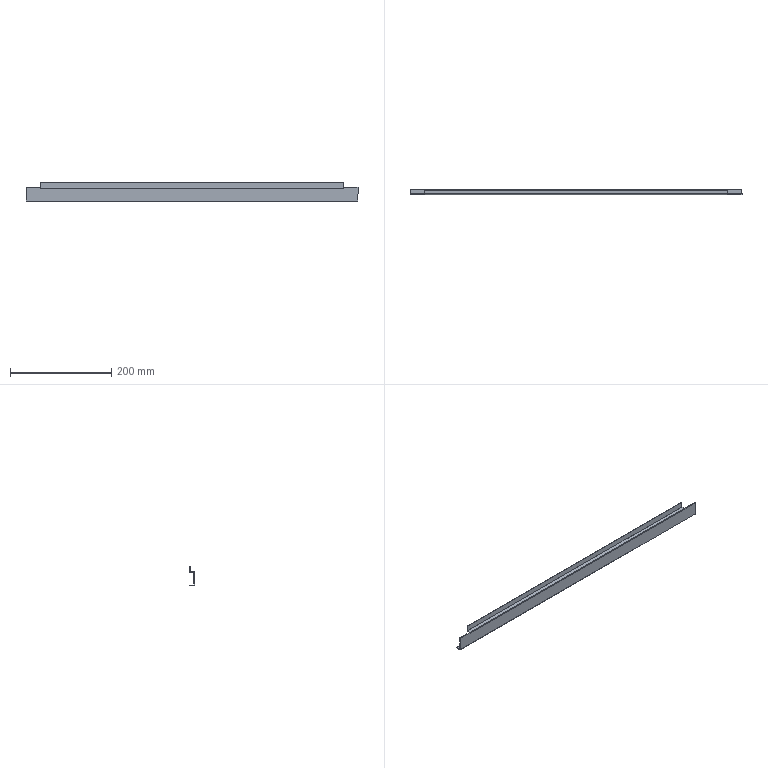Component | SolidWorks | TopCoverRearSideBeam-1 | 1 solid | 40 faces | box 657 x 10 x 39 mm | volume 52545 mm3 | plane 34 | cylinder 6 | commonest cylinder face diameters 0.2 x3 3.2 x3
STEP:
#1=CARTESIAN_POINT('',(10.065,14.168,24.67));
#2=VERTEX_POINT('',#1);
#3=CARTESIAN_POINT('',(10.065,14.168,24.675));
#4=VERTEX_POINT('',#3);
#5=CARTESIAN_POINT('',(10.065,14.168,24.675));
#6=DIRECTION('',(0.,0.,1.));
#7=VECTOR('',#6,39.37);
#8=LINE('',#5,#7);
#9=EDGE_CURVE('',#2,#4,#8,.T.);
#10=ORIENTED_EDGE('',*,*,#9,.F.);
#11=CARTESIAN_POINT('',(10.065,14.164,24.671));
#12=VERTEX_POINT('',#11);
#13=CARTESIAN_POINT('',(10.065,14.164,24.67));
#14=DIRECTION('',(-0.,-1.,0.));
#15=VECTOR('',#14,39.37);
#16=LINE('',#13,#15);
#17=EDGE_CURVE('',#2,#12,#16,.T.);
#18=ORIENTED_EDGE('',*,*,#17,.T.);
#19=CARTESIAN_POINT('',(10.065,14.164,24.612));
#20=VERTEX_POINT('',#19);
#21=CARTESIAN_POINT('',(10.065,14.164,24.671));
#22=DIRECTION('',(-0.,-0.,-1.));
#23=VECTOR('',#22,39.37);
#24=LINE('',#21,#23);
#25=EDGE_CURVE('',#12,#20,#24,.T.);
#26=ORIENTED_EDGE('',*,*,#25,.T.);
#27=CARTESIAN_POINT('',(10.065,14.227,24.675));
#28=VERTEX_POINT('',#27);
#29=CARTESIAN_POINT('',(10.065,14.164,24.675));
#30=DIRECTION('',(1.,-0.,-0.));
#31=DIRECTION('',(0.,1.,0.));
#32=AXIS2_PLACEMENT_3D('',#29,#30,#31);
#33=CIRCLE('',#32,0.06299);
#34=EDGE_CURVE('',#20,#28,#33,.T.);
#35=ORIENTED_EDGE('',*,*,#34,.T.);
#36=CARTESIAN_POINT('',(10.065,14.227,24.675));
#37=DIRECTION('',(0.,1.,-0.));
#38=VECTOR('',#37,39.37);
#39=LINE('',#36,#38);
#40=EDGE_CURVE('',#4,#28,#39,.T.);
#41=ORIENTED_EDGE('',*,*,#40,.F.);
#42=EDGE_LOOP('',(#10,#18,#26,#35,#41));
#43=FACE_OUTER_BOUND('',#42,.T.);
#44=CARTESIAN_POINT('',(10.065,14.164,24.675));
#45=DIRECTION('',(1.,-0.,-0.));
#46=DIRECTION('',(-0.,-1.,0.));
#47=AXIS2_PLACEMENT_3D('',#44,#45,#46);
#48=PLANE('',#47);
#49=ADVANCED_FACE('',(#43),#48,.T.);
#50=CARTESIAN_POINT('',(-13.557,14.164,24.671));
#51=VERTEX_POINT('',#50);
#52=CARTESIAN_POINT('',(-13.557,14.164,24.612));
#53=VERTEX_POINT('',#52);
#54=CARTESIAN_POINT('',(-13.557,14.164,24.671));
#55=DIRECTION('',(-0.,-0.,-1.));
#56=VECTOR('',#55,39.37);
#57=LINE('',#54,#56);
#58=EDGE_CURVE('',#51,#53,#57,.T.);
#59=ORIENTED_EDGE('',*,*,#58,.F.);
#60=CARTESIAN_POINT('',(-13.557,14.168,24.67));
#61=VERTEX_POINT('',#60);
#62=CARTESIAN_POINT('',(-13.557,14.164,24.67));
#63=DIRECTION('',(0.,1.,-0.));
#64=VECTOR('',#63,39.37);
#65=LINE('',#62,#64);
#66=EDGE_CURVE('',#51,#61,#65,.T.);
#67=ORIENTED_EDGE('',*,*,#66,.T.);
#68=CARTESIAN_POINT('',(-13.557,14.168,24.675));
#69=VERTEX_POINT('',#68);
#70=CARTESIAN_POINT('',(-13.557,14.168,24.675));
#71=DIRECTION('',(-0.,-0.,-1.));
#72=VECTOR('',#71,39.37);
#73=LINE('',#70,#72);
#74=EDGE_CURVE('',#69,#61,#73,.T.);
#75=ORIENTED_EDGE('',*,*,#74,.F.);
#76=CARTESIAN_POINT('',(-13.557,14.227,24.675));
#77=VERTEX_POINT('',#76);
#78=CARTESIAN_POINT('',(-13.557,14.168,24.675));
#79=DIRECTION('',(0.,1.,-0.));
#80=VECTOR('',#79,39.37);
#81=LINE('',#78,#80);
#82=EDGE_CURVE('',#69,#77,#81,.T.);
#83=ORIENTED_EDGE('',*,*,#82,.T.);
#84=CARTESIAN_POINT('',(-13.557,14.164,24.675));
#85=DIRECTION('',(-1.,0.,0.));
#86=DIRECTION('',(0.,1.,0.));
#87=AXIS2_PLACEMENT_3D('',#84,#85,#86);
#88=CIRCLE('',#87,0.06299);
#89=EDGE_CURVE('',#77,#53,#88,.T.);
#90=ORIENTED_EDGE('',*,*,#89,.T.);
#91=EDGE_LOOP('',(#59,#67,#75,#83,#90));
#92=FACE_OUTER_BOUND('',#91,.T.);
#93=CARTESIAN_POINT('',(-13.557,14.164,24.675));
#94=DIRECTION('',(1.,-0.,-0.));
#95=DIRECTION('',(-0.,-1.,0.));
#96=AXIS2_PLACEMENT_3D('',#93,#94,#95);
#97=PLANE('',#96);
#98=ADVANCED_FACE('',(#92),#97,.F.);
#99=CARTESIAN_POINT('',(9.982,14.168,24.675));
#100=VERTEX_POINT('',#99);
#101=CARTESIAN_POINT('',(9.982,14.164,24.671));
#102=VERTEX_POINT('',#101);
#103=CARTESIAN_POINT('',(9.982,14.164,24.675));
#104=DIRECTION('',(-1.,0.,0.));
#105=DIRECTION('',(0.,-1.,0.));
#106=AXIS2_PLACEMENT_3D('',#103,#104,#105);
#107=CIRCLE('',#106,0.003937);
#108=EDGE_CURVE('',#100,#102,#107,.T.);
#109=ORIENTED_EDGE('',*,*,#108,.F.);
#110=CARTESIAN_POINT('',(-13.475,14.168,24.675));
#111=VERTEX_POINT('',#110);
#112=CARTESIAN_POINT('',(10.065,14.168,24.675));
#113=DIRECTION('',(-1.,0.,0.));
#114=VECTOR('',#113,39.37);
#115=LINE('',#112,#114);
#116=EDGE_CURVE('',#100,#111,#115,.T.);
#117=ORIENTED_EDGE('',*,*,#116,.T.);
#118=CARTESIAN_POINT('',(-13.475,14.164,24.671));
#119=VERTEX_POINT('',#118);
#120=CARTESIAN_POINT('',(-13.475,14.164,24.675));
#121=DIRECTION('',(1.,-0.,-0.));
#122=DIRECTION('',(0.,1.,-0.));
#123=AXIS2_PLACEMENT_3D('',#120,#121,#122);
#124=CIRCLE('',#123,0.003937);
#125=EDGE_CURVE('',#119,#111,#124,.T.);
#126=ORIENTED_EDGE('',*,*,#125,.F.);
#127=CARTESIAN_POINT('',(-13.557,14.164,24.671));
#128=DIRECTION('',(1.,-0.,-0.));
#129=VECTOR('',#128,39.37);
#130=LINE('',#127,#129);
#131=EDGE_CURVE('',#119,#102,#130,.T.);
#132=ORIENTED_EDGE('',*,*,#131,.T.);
#133=EDGE_LOOP('',(#109,#117,#126,#132));
#134=FACE_OUTER_BOUND('',#133,.T.);
#135=CARTESIAN_POINT('',(-13.557,14.164,24.675));
#136=DIRECTION('',(-1.,0.,0.));
#137=DIRECTION('',(0.,1.,0.));
#138=AXIS2_PLACEMENT_3D('',#135,#136,#137);
#139=CYLINDRICAL_SURFACE('',#138,0.003937);
#140=ADVANCED_FACE('',(#134),#139,.F.);
#141=ORIENTED_EDGE('',*,*,#58,.T.);
#142=CARTESIAN_POINT('',(-13.557,13.896,24.612));
#143=VERTEX_POINT('',#142);
#144=CARTESIAN_POINT('',(-13.557,13.892,24.612));
#145=DIRECTION('',(-0.,-1.,-0.));
#146=VECTOR('',#145,39.37);
#147=LINE('',#144,#146);
#148=EDGE_CURVE('',#53,#143,#147,.T.);
#149=ORIENTED_EDGE('',*,*,#148,.T.);
#150=CARTESIAN_POINT('',(-13.557,13.896,24.671));
#151=VERTEX_POINT('',#150);
#152=CARTESIAN_POINT('',(-13.557,13.896,24.671));
#153=DIRECTION('',(0.,-0.,1.));
#154=VECTOR('',#153,39.37);
#155=LINE('',#152,#154);
#156=EDGE_CURVE('',#143,#151,#155,.T.);
#157=ORIENTED_EDGE('',*,*,#156,.T.);
#158=CARTESIAN_POINT('',(-13.557,13.892,24.671));
#159=DIRECTION('',(-0.,-1.,-0.));
#160=VECTOR('',#159,39.37);
#161=LINE('',#158,#160);
#162=EDGE_CURVE('',#51,#151,#161,.T.);
#163=ORIENTED_EDGE('',*,*,#162,.F.);
#164=EDGE_LOOP('',(#141,#149,#157,#163));
#165=FACE_OUTER_BOUND('',#164,.T.);
#166=CARTESIAN_POINT('',(-13.557,13.892,24.671));
#167=DIRECTION('',(1.,-0.,-0.));
#168=DIRECTION('',(-0.,-1.,0.));
#169=AXIS2_PLACEMENT_3D('',#166,#167,#168);
#170=PLANE('',#169);
#171=ADVANCED_FACE('',(#165),#170,.F.);
#172=ORIENTED_EDGE('',*,*,#25,.F.);
#173=CARTESIAN_POINT('',(10.065,13.896,24.671));
#174=VERTEX_POINT('',#173);
#175=CARTESIAN_POINT('',(10.065,13.892,24.671));
#176=DIRECTION('',(0.,1.,0.));
#177=VECTOR('',#176,39.37);
#178=LINE('',#175,#177);
#179=EDGE_CURVE('',#174,#12,#178,.T.);
#180=ORIENTED_EDGE('',*,*,#179,.F.);
#181=CARTESIAN_POINT('',(10.065,13.896,24.612));
#182=VERTEX_POINT('',#181);
#183=CARTESIAN_POINT('',(10.065,13.896,24.612));
#184=DIRECTION('',(0.,-0.,1.));
#185=VECTOR('',#184,39.37);
#186=LINE('',#183,#185);
#187=EDGE_CURVE('',#182,#174,#186,.T.);
#188=ORIENTED_EDGE('',*,*,#187,.F.);
#189=CARTESIAN_POINT('',(10.065,14.227,24.612));
#190=DIRECTION('',(0.,1.,0.));
#191=VECTOR('',#190,39.37);
#192=LINE('',#189,#191);
#193=EDGE_CURVE('',#182,#20,#192,.T.);
#194=ORIENTED_EDGE('',*,*,#193,.T.);
#195=EDGE_LOOP('',(#172,#180,#188,#194));
#196=FACE_OUTER_BOUND('',#195,.T.);
#197=CARTESIAN_POINT('',(10.065,14.227,24.671));
#198=DIRECTION('',(-1.,0.,0.));
#199=DIRECTION('',(0.,1.,-0.));
#200=AXIS2_PLACEMENT_3D('',#197,#198,#199);
#201=PLANE('',#200);
#202=ADVANCED_FACE('',(#196),#201,.F.);
#203=ORIENTED_EDGE('',*,*,#162,.T.);
#204=CARTESIAN_POINT('',(-13.557,13.896,24.671));
#205=DIRECTION('',(-1.,0.,0.));
#206=VECTOR('',#205,39.37);
#207=LINE('',#204,#206);
#208=EDGE_CURVE('',#174,#151,#207,.T.);
#209=ORIENTED_EDGE('',*,*,#208,.F.);
#210=ORIENTED_EDGE('',*,*,#179,.T.);
#211=CARTESIAN_POINT('',(9.982,14.164,24.671));
#212=CARTESIAN_POINT('',(10.009,14.164,24.67));
#213=CARTESIAN_POINT('',(10.037,14.164,24.67));
#214=CARTESIAN_POINT('',(10.065,14.164,24.671));
#215=B_SPLINE_CURVE_WITH_KNOTS('',3,(#211,#212,#213,#214),.UNSPECIFIED.,.F.,.F.,(4,4),(0.9965,1.),.UNSPECIFIED.);
#216=EDGE_CURVE('',#102,#12,#215,.T.);
#217=ORIENTED_EDGE('',*,*,#216,.F.);
#218=ORIENTED_EDGE('',*,*,#131,.F.);
#219=CARTESIAN_POINT('',(-13.557,14.164,24.671));
#220=CARTESIAN_POINT('',(-13.53,14.164,24.67));
#221=CARTESIAN_POINT('',(-13.502,14.164,24.67));
#222=CARTESIAN_POINT('',(-13.475,14.164,24.671));
#223=B_SPLINE_CURVE_WITH_KNOTS('',3,(#219,#220,#221,#222),.UNSPECIFIED.,.F.,.F.,(4,4),(0.,0.0035),.UNSPECIFIED.);
#224=EDGE_CURVE('',#51,#119,#223,.T.);
#225=ORIENTED_EDGE('',*,*,#224,.F.);
#226=EDGE_LOOP('',(#203,#209,#210,#217,#218,#225));
#227=FACE_OUTER_BOUND('',#226,.T.);
#228=CARTESIAN_POINT('',(-1.746,13.892,24.671));
#229=DIRECTION('',(-0.,0.,-1.));
#230=DIRECTION('',(0.,1.,0.));
#231=AXIS2_PLACEMENT_3D('',#228,#229,#230);
#232=PLANE('',#231);
#233=ADVANCED_FACE('',(#227),#232,.F.);
#234=ORIENTED_EDGE('',*,*,#148,.F.);
#235=CARTESIAN_POINT('',(-13.557,14.164,24.612));
#236=DIRECTION('',(1.,-0.,-0.));
#237=VECTOR('',#236,39.37);
#238=LINE('',#235,#237);
#239=EDGE_CURVE('',#53,#20,#238,.T.);
#240=ORIENTED_EDGE('',*,*,#239,.T.);
#241=ORIENTED_EDGE('',*,*,#193,.F.);
#242=CARTESIAN_POINT('',(-13.557,13.896,24.612));
#243=DIRECTION('',(1.,-0.,-0.));
#244=VECTOR('',#243,39.37);
#245=LINE('',#242,#244);
#246=EDGE_CURVE('',#143,#182,#245,.T.);
#247=ORIENTED_EDGE('',*,*,#246,.F.);
#248=EDGE_LOOP('',(#234,#240,#241,#247));
#249=FACE_OUTER_BOUND('',#248,.T.);
#250=CARTESIAN_POINT('',(-1.746,13.892,24.612));
#251=DIRECTION('',(-0.,0.,-1.));
#252=DIRECTION('',(0.,1.,0.));
#253=AXIS2_PLACEMENT_3D('',#250,#251,#252);
#254=PLANE('',#253);
#255=ADVANCED_FACE('',(#249),#254,.T.);
#256=CARTESIAN_POINT('',(-14.68,13.833,23.612));
#257=VERTEX_POINT('',#256);
#258=CARTESIAN_POINT('',(-14.68,13.833,24.671));
#259=VERTEX_POINT('',#258);
#260=CARTESIAN_POINT('',(-14.68,13.833,24.671));
#261=DIRECTION('',(0.,0.,1.));
#262=VECTOR('',#261,39.37);
#263=LINE('',#260,#262);
#264=EDGE_CURVE('',#257,#259,#263,.T.);
#265=ORIENTED_EDGE('',*,*,#264,.F.);
#266=CARTESIAN_POINT('',(11.187,13.833,23.612));
#267=VERTEX_POINT('',#266);
#268=CARTESIAN_POINT('',(-14.68,13.833,23.612));
#269=DIRECTION('',(1.,-0.,-0.));
#270=VECTOR('',#269,39.37);
#271=LINE('',#268,#270);
#272=EDGE_CURVE('',#257,#267,#271,.T.);
#273=ORIENTED_EDGE('',*,*,#272,.T.);
#274=CARTESIAN_POINT('',(11.187,13.833,24.671));
#275=VERTEX_POINT('',#274);
#276=CARTESIAN_POINT('',(11.187,13.833,24.671));
#277=DIRECTION('',(-0.,-0.,-1.));
#278=VECTOR('',#277,39.37);
#279=LINE('',#276,#278);
#280=EDGE_CURVE('',#275,#267,#279,.T.);
#281=ORIENTED_EDGE('',*,*,#280,.F.);
#282=CARTESIAN_POINT('',(10.065,13.833,24.671));
#283=VERTEX_POINT('',#282);
#284=CARTESIAN_POINT('',(-14.68,13.833,24.671));
#285=DIRECTION('',(1.,-0.,-0.));
#286=VECTOR('',#285,39.37);
#287=LINE('',#284,#286);
#288=EDGE_CURVE('',#283,#275,#287,.T.);
#289=ORIENTED_EDGE('',*,*,#288,.F.);
#290=CARTESIAN_POINT('',(10.065,13.833,24.608));
#291=VERTEX_POINT('',#290);
#292=CARTESIAN_POINT('',(10.065,13.833,24.11));
#293=DIRECTION('',(-0.,-0.,-1.));
#294=VECTOR('',#293,39.37);
#295=LINE('',#292,#294);
#296=EDGE_CURVE('',#283,#291,#295,.T.);
#297=ORIENTED_EDGE('',*,*,#296,.T.);
#298=CARTESIAN_POINT('',(-13.557,13.833,24.608));
#299=VERTEX_POINT('',#298);
#300=CARTESIAN_POINT('',(10.065,13.833,24.608));
#301=DIRECTION('',(-1.,0.,0.));
#302=VECTOR('',#301,39.37);
#303=LINE('',#300,#302);
#304=EDGE_CURVE('',#291,#299,#303,.T.);
#305=ORIENTED_EDGE('',*,*,#304,.T.);
#306=CARTESIAN_POINT('',(-13.557,13.833,24.671));
#307=VERTEX_POINT('',#306);
#308=CARTESIAN_POINT('',(-13.557,13.833,24.11));
#309=DIRECTION('',(0.,0.,1.));
#310=VECTOR('',#309,39.37);
#311=LINE('',#308,#310);
#312=EDGE_CURVE('',#299,#307,#311,.T.);
#313=ORIENTED_EDGE('',*,*,#312,.T.);
#314=CARTESIAN_POINT('',(-14.68,13.833,24.671));
#315=DIRECTION('',(1.,-0.,-0.));
#316=VECTOR('',#315,39.37);
#317=LINE('',#314,#316);
#318=EDGE_CURVE('',#259,#307,#317,.T.);
#319=ORIENTED_EDGE('',*,*,#318,.F.);
#320=EDGE_LOOP('',(#265,#273,#281,#289,#297,#305,#313,#319));
#321=FACE_OUTER_BOUND('',#320,.T.);
#322=CARTESIAN_POINT('',(-1.746,13.833,24.11));
#323=DIRECTION('',(-0.,-1.,0.));
#324=DIRECTION('',(-1.,0.,0.));
#325=AXIS2_PLACEMENT_3D('',#322,#323,#324);
#326=PLANE('',#325);
#327=ADVANCED_FACE('',(#321),#326,.T.);
#328=CARTESIAN_POINT('',(-14.68,13.892,23.612));
#329=VERTEX_POINT('',#328);
#330=CARTESIAN_POINT('',(11.187,13.892,23.612));
#331=VERTEX_POINT('',#330);
#332=CARTESIAN_POINT('',(-14.68,13.892,23.612));
#333=DIRECTION('',(1.,-0.,-0.));
#334=VECTOR('',#333,39.37);
#335=LINE('',#332,#334);
#336=EDGE_CURVE('',#329,#331,#335,.T.);
#337=ORIENTED_EDGE('',*,*,#336,.F.);
#338=CARTESIAN_POINT('',(-14.68,13.892,24.671));
#339=VERTEX_POINT('',#338);
#340=CARTESIAN_POINT('',(-14.68,13.892,24.671));
#341=DIRECTION('',(0.,0.,1.));
#342=VECTOR('',#341,39.37);
#343=LINE('',#340,#342);
#344=EDGE_CURVE('',#329,#339,#343,.T.);
#345=ORIENTED_EDGE('',*,*,#344,.T.);
#346=CARTESIAN_POINT('',(-13.557,13.892,24.671));
#347=VERTEX_POINT('',#346);
#348=CARTESIAN_POINT('',(-14.68,13.892,24.671));
#349=DIRECTION('',(1.,-0.,-0.));
#350=VECTOR('',#349,39.37);
#351=LINE('',#348,#350);
#352=EDGE_CURVE('',#339,#347,#351,.T.);
#353=ORIENTED_EDGE('',*,*,#352,.T.);
#354=CARTESIAN_POINT('',(-13.557,13.892,24.671));
#355=VERTEX_POINT('',#354);
#356=CARTESIAN_POINT('',(-13.557,13.892,24.608));
#357=DIRECTION('',(0.,-0.,1.));
#358=VECTOR('',#357,39.37);
#359=LINE('',#356,#358);
#360=EDGE_CURVE('',#355,#347,#359,.T.);
#361=ORIENTED_EDGE('',*,*,#360,.F.);
#362=CARTESIAN_POINT('',(-13.557,13.892,24.608));
#363=VERTEX_POINT('',#362);
#364=CARTESIAN_POINT('',(-13.557,13.892,24.608));
#365=DIRECTION('',(0.,-0.,1.));
#366=VECTOR('',#365,39.37);
#367=LINE('',#364,#366);
#368=EDGE_CURVE('',#363,#355,#367,.T.);
#369=ORIENTED_EDGE('',*,*,#368,.F.);
#370=CARTESIAN_POINT('',(10.065,13.892,24.608));
#371=VERTEX_POINT('',#370);
#372=CARTESIAN_POINT('',(10.065,13.892,24.608));
#373=DIRECTION('',(-1.,0.,0.));
#374=VECTOR('',#373,39.37);
#375=LINE('',#372,#374);
#376=EDGE_CURVE('',#371,#363,#375,.T.);
#377=ORIENTED_EDGE('',*,*,#376,.F.);
#378=CARTESIAN_POINT('',(10.065,13.892,24.671));
#379=VERTEX_POINT('',#378);
#380=CARTESIAN_POINT('',(10.065,13.892,24.671));
#381=DIRECTION('',(-0.,0.,-1.));
#382=VECTOR('',#381,39.37);
#383=LINE('',#380,#382);
#384=EDGE_CURVE('',#379,#371,#383,.T.);
#385=ORIENTED_EDGE('',*,*,#384,.F.);
#386=CARTESIAN_POINT('',(10.065,13.892,24.671));
#387=VERTEX_POINT('',#386);
#388=CARTESIAN_POINT('',(10.065,13.892,24.671));
#389=DIRECTION('',(-0.,0.,-1.));
#390=VECTOR('',#389,39.37);
#391=LINE('',#388,#390);
#392=EDGE_CURVE('',#387,#379,#391,.T.);
#393=ORIENTED_EDGE('',*,*,#392,.F.);
#394=CARTESIAN_POINT('',(11.187,13.892,24.671));
#395=VERTEX_POINT('',#394);
#396=CARTESIAN_POINT('',(-14.68,13.892,24.671));
#397=DIRECTION('',(1.,-0.,-0.));
#398=VECTOR('',#397,39.37);
#399=LINE('',#396,#398);
#400=EDGE_CURVE('',#387,#395,#399,.T.);
#401=ORIENTED_EDGE('',*,*,#400,.T.);
#402=CARTESIAN_POINT('',(11.187,13.892,24.671));
#403=DIRECTION('',(-0.,-0.,-1.));
#404=VECTOR('',#403,39.37);
#405=LINE('',#402,#404);
#406=EDGE_CURVE('',#395,#331,#405,.T.);
#407=ORIENTED_EDGE('',*,*,#406,.T.);
#408=EDGE_LOOP('',(#337,#345,#353,#361,#369,#377,#385,#393,#401,#407));
#409=FACE_OUTER_BOUND('',#408,.T.);
#410=CARTESIAN_POINT('',(-1.746,13.892,24.11));
#411=DIRECTION('',(-0.,-1.,0.));
#412=DIRECTION('',(-1.,0.,0.));
#413=AXIS2_PLACEMENT_3D('',#410,#411,#412);
#414=PLANE('',#413);
#415=ADVANCED_FACE('',(#409),#414,.F.);
#416=ORIENTED_EDGE('',*,*,#344,.F.);
#417=CARTESIAN_POINT('',(-14.68,13.892,23.612));
#418=DIRECTION('',(-0.,-1.,0.));
#419=VECTOR('',#418,39.37);
#420=LINE('',#417,#419);
#421=EDGE_CURVE('',#329,#257,#420,.T.);
#422=ORIENTED_EDGE('',*,*,#421,.T.);
#423=ORIENTED_EDGE('',*,*,#264,.T.);
#424=CARTESIAN_POINT('',(-14.68,13.833,24.671));
#425=DIRECTION('',(0.,1.,-0.));
#426=VECTOR('',#425,39.37);
#427=LINE('',#424,#426);
#428=EDGE_CURVE('',#259,#339,#427,.T.);
#429=ORIENTED_EDGE('',*,*,#428,.T.);
#430=EDGE_LOOP('',(#416,#422,#423,#429));
#431=FACE_OUTER_BOUND('',#430,.T.);
#432=CARTESIAN_POINT('',(-14.68,13.833,24.671));
#433=DIRECTION('',(-1.,0.,0.));
#434=DIRECTION('',(0.,1.,-0.));
#435=AXIS2_PLACEMENT_3D('',#432,#433,#434);
#436=PLANE('',#435);
#437=ADVANCED_FACE('',(#431),#436,.T.);
#438=ORIENTED_EDGE('',*,*,#392,.T.);
#439=CARTESIAN_POINT('',(10.065,13.896,24.608));
#440=DIRECTION('',(1.,-0.,-0.));
#441=DIRECTION('',(0.,-1.,0.));
#442=AXIS2_PLACEMENT_3D('',#439,#440,#441);
#443=CIRCLE('',#442,0.06299);
#444=EDGE_CURVE('',#379,#291,#443,.T.);
#445=ORIENTED_EDGE('',*,*,#444,.T.);
#446=ORIENTED_EDGE('',*,*,#296,.F.);
#447=CARTESIAN_POINT('',(10.065,13.892,24.671));
#448=DIRECTION('',(-0.,-1.,-0.));
#449=VECTOR('',#448,39.37);
#450=LINE('',#447,#449);
#451=EDGE_CURVE('',#387,#283,#450,.T.);
#452=ORIENTED_EDGE('',*,*,#451,.F.);
#453=EDGE_LOOP('',(#438,#445,#446,#452));
#454=FACE_OUTER_BOUND('',#453,.T.);
#455=CARTESIAN_POINT('',(10.065,13.892,24.671));
#456=DIRECTION('',(-1.,0.,0.));
#457=DIRECTION('',(0.,1.,-0.));
#458=AXIS2_PLACEMENT_3D('',#455,#456,#457);
#459=PLANE('',#458);
#460=ADVANCED_FACE('',(#454),#459,.T.);
#461=ORIENTED_EDGE('',*,*,#312,.F.);
#462=CARTESIAN_POINT('',(-13.557,13.896,24.608));
#463=DIRECTION('',(-1.,0.,0.));
#464=DIRECTION('',(0.,-1.,0.));
#465=AXIS2_PLACEMENT_3D('',#462,#463,#464);
#466=CIRCLE('',#465,0.06299);
#467=EDGE_CURVE('',#299,#355,#466,.T.);
#468=ORIENTED_EDGE('',*,*,#467,.T.);
#469=ORIENTED_EDGE('',*,*,#360,.T.);
#470=CARTESIAN_POINT('',(-13.557,13.892,24.671));
#471=DIRECTION('',(-0.,-1.,-0.));
#472=VECTOR('',#471,39.37);
#473=LINE('',#470,#472);
#474=EDGE_CURVE('',#347,#307,#473,.T.);
#475=ORIENTED_EDGE('',*,*,#474,.T.);
#476=EDGE_LOOP('',(#461,#468,#469,#475));
#477=FACE_OUTER_BOUND('',#476,.T.);
#478=CARTESIAN_POINT('',(-13.557,13.892,24.608));
#479=DIRECTION('',(1.,-0.,-0.));
#480=DIRECTION('',(-0.,-1.,0.));
#481=AXIS2_PLACEMENT_3D('',#478,#479,#480);
#482=PLANE('',#481);
#483=ADVANCED_FACE('',(#477),#482,.T.);
#484=ORIENTED_EDGE('',*,*,#400,.F.);
#485=ORIENTED_EDGE('',*,*,#451,.T.);
#486=ORIENTED_EDGE('',*,*,#288,.T.);
#487=CARTESIAN_POINT('',(11.187,13.833,24.671));
#488=DIRECTION('',(0.,1.,-0.));
#489=VECTOR('',#488,39.37);
#490=LINE('',#487,#489);
#491=EDGE_CURVE('',#275,#395,#490,.T.);
#492=ORIENTED_EDGE('',*,*,#491,.T.);
#493=EDGE_LOOP('',(#484,#485,#486,#492));
#494=FACE_OUTER_BOUND('',#493,.T.);
#495=CARTESIAN_POINT('',(-14.68,13.833,24.671));
#496=DIRECTION('',(0.,0.,1.));
#497=DIRECTION('',(-0.,-1.,0.));
#498=AXIS2_PLACEMENT_3D('',#495,#496,#497);
#499=PLANE('',#498);
#500=ADVANCED_FACE('',(#494),#499,.T.);
#501=ORIENTED_EDGE('',*,*,#318,.T.);
#502=ORIENTED_EDGE('',*,*,#474,.F.);
#503=ORIENTED_EDGE('',*,*,#352,.F.);
#504=ORIENTED_EDGE('',*,*,#428,.F.);
#505=EDGE_LOOP('',(#501,#502,#503,#504));
#506=FACE_OUTER_BOUND('',#505,.T.);
#507=CARTESIAN_POINT('',(-14.68,13.833,24.671));
#508=DIRECTION('',(0.,0.,1.));
#509=DIRECTION('',(-0.,-1.,0.));
#510=AXIS2_PLACEMENT_3D('',#507,#508,#509);
#511=PLANE('',#510);
#512=ADVANCED_FACE('',(#506),#511,.T.);
#513=CARTESIAN_POINT('',(11.187,13.892,23.612));
#514=DIRECTION('',(-0.,-1.,0.));
#515=VECTOR('',#514,39.37);
#516=LINE('',#513,#515);
#517=EDGE_CURVE('',#331,#267,#516,.T.);
#518=ORIENTED_EDGE('',*,*,#517,.F.);
#519=ORIENTED_EDGE('',*,*,#406,.F.);
#520=ORIENTED_EDGE('',*,*,#491,.F.);
#521=ORIENTED_EDGE('',*,*,#280,.T.);
#522=EDGE_LOOP('',(#518,#519,#520,#521));
#523=FACE_OUTER_BOUND('',#522,.T.);
#524=CARTESIAN_POINT('',(11.187,13.833,24.671));
#525=DIRECTION('',(1.,-0.,-0.));
#526=DIRECTION('',(-0.,-1.,0.));
#527=AXIS2_PLACEMENT_3D('',#524,#525,#526);
#528=PLANE('',#527);
#529=ADVANCED_FACE('',(#523),#528,.T.);
#530=CARTESIAN_POINT('',(-13.557,13.896,24.608));
#531=DIRECTION('',(-1.,0.,0.));
#532=DIRECTION('',(0.,-1.,0.));
#533=AXIS2_PLACEMENT_3D('',#530,#531,#532);
#534=CIRCLE('',#533,0.003937);
#535=EDGE_CURVE('',#363,#143,#534,.T.);
#536=ORIENTED_EDGE('',*,*,#535,.F.);
#537=ORIENTED_EDGE('',*,*,#368,.T.);
#538=CARTESIAN_POINT('',(-13.557,13.896,24.608));
#539=DIRECTION('',(-1.,0.,0.));
#540=DIRECTION('',(0.,-1.,0.));
#541=AXIS2_PLACEMENT_3D('',#538,#539,#540);
#542=CIRCLE('',#541,0.06299);
#543=EDGE_CURVE('',#355,#151,#542,.T.);
#544=ORIENTED_EDGE('',*,*,#543,.T.);
#545=ORIENTED_EDGE('',*,*,#156,.F.);
#546=EDGE_LOOP('',(#536,#537,#544,#545));
#547=FACE_OUTER_BOUND('',#546,.T.);
#548=CARTESIAN_POINT('',(-13.557,13.896,24.608));
#549=DIRECTION('',(-1.,0.,0.));
#550=DIRECTION('',(0.,1.,-0.));
#551=AXIS2_PLACEMENT_3D('',#548,#549,#550);
#552=PLANE('',#551);
#553=ADVANCED_FACE('',(#547),#552,.T.);
#554=CARTESIAN_POINT('',(10.065,13.896,24.608));
#555=DIRECTION('',(1.,-0.,-0.));
#556=DIRECTION('',(0.,-1.,0.));
#557=AXIS2_PLACEMENT_3D('',#554,#555,#556);
#558=CIRCLE('',#557,0.06299);
#559=EDGE_CURVE('',#174,#379,#558,.T.);
#560=ORIENTED_EDGE('',*,*,#559,.T.);
#561=ORIENTED_EDGE('',*,*,#384,.T.);
#562=CARTESIAN_POINT('',(10.065,13.896,24.608));
#563=DIRECTION('',(1.,-0.,-0.));
#564=DIRECTION('',(0.,-1.,0.));
#565=AXIS2_PLACEMENT_3D('',#562,#563,#564);
#566=CIRCLE('',#565,0.003937);
#567=EDGE_CURVE('',#182,#371,#566,.T.);
#568=ORIENTED_EDGE('',*,*,#567,.F.);
#569=ORIENTED_EDGE('',*,*,#187,.T.);
#570=EDGE_LOOP('',(#560,#561,#568,#569));
#571=FACE_OUTER_BOUND('',#570,.T.);
#572=CARTESIAN_POINT('',(10.065,13.896,24.608));
#573=DIRECTION('',(-1.,0.,0.));
#574=DIRECTION('',(0.,1.,-0.));
#575=AXIS2_PLACEMENT_3D('',#572,#573,#574);
#576=PLANE('',#575);
#577=ADVANCED_FACE('',(#571),#576,.F.);
#578=ORIENTED_EDGE('',*,*,#304,.F.);
#579=ORIENTED_EDGE('',*,*,#444,.F.);
#580=ORIENTED_EDGE('',*,*,#559,.F.);
#581=ORIENTED_EDGE('',*,*,#208,.T.);
#582=ORIENTED_EDGE('',*,*,#543,.F.);
#583=ORIENTED_EDGE('',*,*,#467,.F.);
#584=EDGE_LOOP('',(#578,#579,#580,#581,#582,#583));
#585=FACE_OUTER_BOUND('',#584,.T.);
#586=CARTESIAN_POINT('',(10.065,13.896,24.608));
#587=DIRECTION('',(1.,-0.,-0.));
#588=DIRECTION('',(0.,0.,1.));
#589=AXIS2_PLACEMENT_3D('',#586,#587,#588);
#590=CYLINDRICAL_SURFACE('',#589,0.06299);
#591=ADVANCED_FACE('',(#585),#590,.T.);
#592=ORIENTED_EDGE('',*,*,#376,.T.);
#593=ORIENTED_EDGE('',*,*,#535,.T.);
#594=ORIENTED_EDGE('',*,*,#246,.T.);
#595=ORIENTED_EDGE('',*,*,#567,.T.);
#596=EDGE_LOOP('',(#592,#593,#594,#595));
#597=FACE_OUTER_BOUND('',#596,.T.);
#598=CARTESIAN_POINT('',(10.065,13.896,24.608));
#599=DIRECTION('',(1.,-0.,-0.));
#600=DIRECTION('',(0.,0.,1.));
#601=AXIS2_PLACEMENT_3D('',#598,#599,#600);
#602=CYLINDRICAL_SURFACE('',#601,0.003937);
#603=ADVANCED_FACE('',(#597),#602,.F.);
#604=CARTESIAN_POINT('',(11.187,13.896,23.608));
#605=VERTEX_POINT('',#604);
#606=CARTESIAN_POINT('',(11.187,13.896,23.549));
#607=VERTEX_POINT('',#606);
#608=CARTESIAN_POINT('',(11.187,13.896,23.549));
#609=DIRECTION('',(-0.,-0.,-1.));
#610=VECTOR('',#609,39.37);
#611=LINE('',#608,#610);
#612=EDGE_CURVE('',#605,#607,#611,.T.);
#613=ORIENTED_EDGE('',*,*,#612,.F.);
#614=CARTESIAN_POINT('',(11.187,13.896,23.612));
#615=DIRECTION('',(1.,-0.,-0.));
#616=DIRECTION('',(0.,1.,0.));
#617=AXIS2_PLACEMENT_3D('',#614,#615,#616);
#618=CIRCLE('',#617,0.003937);
#619=EDGE_CURVE('',#331,#605,#618,.T.);
#620=ORIENTED_EDGE('',*,*,#619,.F.);
#621=ORIENTED_EDGE('',*,*,#517,.T.);
#622=CARTESIAN_POINT('',(11.187,13.896,23.612));
#623=DIRECTION('',(1.,-0.,-0.));
#624=DIRECTION('',(0.,1.,0.));
#625=AXIS2_PLACEMENT_3D('',#622,#623,#624);
#626=CIRCLE('',#625,0.06299);
#627=EDGE_CURVE('',#267,#607,#626,.T.);
#628=ORIENTED_EDGE('',*,*,#627,.T.);
#629=EDGE_LOOP('',(#613,#620,#621,#628));
#630=FACE_OUTER_BOUND('',#629,.T.);
#631=CARTESIAN_POINT('',(11.187,13.896,23.612));
#632=DIRECTION('',(1.,-0.,-0.));
#633=DIRECTION('',(-0.,-1.,0.));
#634=AXIS2_PLACEMENT_3D('',#631,#632,#633);
#635=PLANE('',#634);
#636=ADVANCED_FACE('',(#630),#635,.T.);
#637=CARTESIAN_POINT('',(-14.68,13.896,23.608));
#638=VERTEX_POINT('',#637);
#639=CARTESIAN_POINT('',(-14.68,13.896,23.612));
#640=DIRECTION('',(-1.,0.,0.));
#641=DIRECTION('',(0.,1.,0.));
#642=AXIS2_PLACEMENT_3D('',#639,#640,#641);
#643=CIRCLE('',#642,0.003937);
#644=EDGE_CURVE('',#638,#329,#643,.T.);
#645=ORIENTED_EDGE('',*,*,#644,.F.);
#646=CARTESIAN_POINT('',(-14.68,13.896,23.549));
#647=VERTEX_POINT('',#646);
#648=CARTESIAN_POINT('',(-14.68,13.896,23.608));
#649=DIRECTION('',(-0.,-0.,-1.));
#650=VECTOR('',#649,39.37);
#651=LINE('',#648,#650);
#652=EDGE_CURVE('',#638,#647,#651,.T.);
#653=ORIENTED_EDGE('',*,*,#652,.T.);
#654=CARTESIAN_POINT('',(-14.68,13.896,23.612));
#655=DIRECTION('',(-1.,0.,0.));
#656=DIRECTION('',(0.,1.,0.));
#657=AXIS2_PLACEMENT_3D('',#654,#655,#656);
#658=CIRCLE('',#657,0.06299);
#659=EDGE_CURVE('',#647,#257,#658,.T.);
#660=ORIENTED_EDGE('',*,*,#659,.T.);
#661=ORIENTED_EDGE('',*,*,#421,.F.);
#662=EDGE_LOOP('',(#645,#653,#660,#661));
#663=FACE_OUTER_BOUND('',#662,.T.);
#664=CARTESIAN_POINT('',(-14.68,13.896,23.612));
#665=DIRECTION('',(1.,-0.,-0.));
#666=DIRECTION('',(-0.,-1.,0.));
#667=AXIS2_PLACEMENT_3D('',#664,#665,#666);
#668=PLANE('',#667);
#669=ADVANCED_FACE('',(#663),#668,.F.);
#670=ORIENTED_EDGE('',*,*,#272,.F.);
#671=ORIENTED_EDGE('',*,*,#659,.F.);
#672=CARTESIAN_POINT('',(-1.746,13.896,23.549));
#673=DIRECTION('',(-1.,0.,0.));
#674=VECTOR('',#673,39.37);
#675=LINE('',#672,#674);
#676=EDGE_CURVE('',#607,#647,#675,.T.);
#677=ORIENTED_EDGE('',*,*,#676,.F.);
#678=ORIENTED_EDGE('',*,*,#627,.F.);
#679=EDGE_LOOP('',(#670,#671,#677,#678));
#680=FACE_OUTER_BOUND('',#679,.T.);
#681=CARTESIAN_POINT('',(-14.68,13.896,23.612));
#682=DIRECTION('',(-1.,0.,0.));
#683=DIRECTION('',(0.,0.,-1.));
#684=AXIS2_PLACEMENT_3D('',#681,#682,#683);
#685=CYLINDRICAL_SURFACE('',#684,0.06299);
#686=ADVANCED_FACE('',(#680),#685,.T.);
#687=ORIENTED_EDGE('',*,*,#336,.T.);
#688=ORIENTED_EDGE('',*,*,#619,.T.);
#689=CARTESIAN_POINT('',(11.187,13.896,23.608));
#690=DIRECTION('',(-1.,0.,0.));
#691=VECTOR('',#690,39.37);
#692=LINE('',#689,#691);
#693=EDGE_CURVE('',#605,#638,#692,.T.);
#694=ORIENTED_EDGE('',*,*,#693,.T.);
#695=ORIENTED_EDGE('',*,*,#644,.T.);
#696=EDGE_LOOP('',(#687,#688,#694,#695));
#697=FACE_OUTER_BOUND('',#696,.T.);
#698=CARTESIAN_POINT('',(-14.68,13.896,23.612));
#699=DIRECTION('',(-1.,0.,0.));
#700=DIRECTION('',(0.,0.,-1.));
#701=AXIS2_PLACEMENT_3D('',#698,#699,#700);
#702=CYLINDRICAL_SURFACE('',#701,0.003937);
#703=ADVANCED_FACE('',(#697),#702,.F.);
#704=CARTESIAN_POINT('',(-14.68,14.227,23.549));
#705=VERTEX_POINT('',#704);
#706=CARTESIAN_POINT('',(-14.68,13.892,23.549));
#707=DIRECTION('',(-0.,-1.,0.));
#708=VECTOR('',#707,39.37);
#709=LINE('',#706,#708);
#710=EDGE_CURVE('',#705,#647,#709,.T.);
#711=ORIENTED_EDGE('',*,*,#710,.T.);
#712=ORIENTED_EDGE('',*,*,#652,.F.);
#713=CARTESIAN_POINT('',(-14.68,14.227,23.608));
#714=VERTEX_POINT('',#713);
#715=CARTESIAN_POINT('',(-14.68,13.892,23.608));
#716=DIRECTION('',(-0.,-1.,0.));
#717=VECTOR('',#716,39.37);
#718=LINE('',#715,#717);
#719=EDGE_CURVE('',#714,#638,#718,.T.);
#720=ORIENTED_EDGE('',*,*,#719,.F.);
#721=CARTESIAN_POINT('',(-14.68,14.227,23.549));
#722=DIRECTION('',(0.,0.,1.));
#723=VECTOR('',#722,39.37);
#724=LINE('',#721,#723);
#725=EDGE_CURVE('',#705,#714,#724,.T.);
#726=ORIENTED_EDGE('',*,*,#725,.F.);
#727=EDGE_LOOP('',(#711,#712,#720,#726));
#728=FACE_OUTER_BOUND('',#727,.T.);
#729=CARTESIAN_POINT('',(-14.68,13.892,23.549));
#730=DIRECTION('',(-1.,0.,0.));
#731=DIRECTION('',(0.,1.,-0.));
#732=AXIS2_PLACEMENT_3D('',#729,#730,#731);
#733=PLANE('',#732);
#734=ADVANCED_FACE('',(#728),#733,.T.);
#735=CARTESIAN_POINT('',(11.187,14.227,23.608));
#736=VERTEX_POINT('',#735);
#737=CARTESIAN_POINT('',(11.187,13.892,23.608));
#738=DIRECTION('',(0.,1.,-0.));
#739=VECTOR('',#738,39.37);
#740=LINE('',#737,#739);
#741=EDGE_CURVE('',#605,#736,#740,.T.);
#742=ORIENTED_EDGE('',*,*,#741,.F.);
#743=ORIENTED_EDGE('',*,*,#612,.T.);
#744=CARTESIAN_POINT('',(11.187,14.227,23.549));
#745=VERTEX_POINT('',#744);
#746=CARTESIAN_POINT('',(11.187,14.227,23.549));
#747=DIRECTION('',(0.,1.,-0.));
#748=VECTOR('',#747,39.37);
#749=LINE('',#746,#748);
#750=EDGE_CURVE('',#607,#745,#749,.T.);
#751=ORIENTED_EDGE('',*,*,#750,.T.);
#752=CARTESIAN_POINT('',(11.187,14.227,23.549));
#753=DIRECTION('',(0.,0.,1.));
#754=VECTOR('',#753,39.37);
#755=LINE('',#752,#754);
#756=EDGE_CURVE('',#745,#736,#755,.T.);
#757=ORIENTED_EDGE('',*,*,#756,.T.);
#758=EDGE_LOOP('',(#742,#743,#751,#757));
#759=FACE_OUTER_BOUND('',#758,.T.);
#760=CARTESIAN_POINT('',(11.187,14.227,23.549));
#761=DIRECTION('',(1.,-0.,-0.));
#762=DIRECTION('',(-0.,-1.,0.));
#763=AXIS2_PLACEMENT_3D('',#760,#761,#762);
#764=PLANE('',#763);
#765=ADVANCED_FACE('',(#759),#764,.T.);
#766=ORIENTED_EDGE('',*,*,#750,.F.);
#767=ORIENTED_EDGE('',*,*,#676,.T.);
#768=ORIENTED_EDGE('',*,*,#710,.F.);
#769=CARTESIAN_POINT('',(-14.68,14.227,23.549));
#770=DIRECTION('',(-1.,0.,0.));
#771=VECTOR('',#770,39.37);
#772=LINE('',#769,#771);
#773=EDGE_CURVE('',#745,#705,#772,.T.);
#774=ORIENTED_EDGE('',*,*,#773,.F.);
#775=EDGE_LOOP('',(#766,#767,#768,#774));
#776=FACE_OUTER_BOUND('',#775,.T.);
#777=CARTESIAN_POINT('',(-1.746,13.892,23.549));
#778=DIRECTION('',(-0.,-0.,-1.));
#779=DIRECTION('',(0.,1.,-0.));
#780=AXIS2_PLACEMENT_3D('',#777,#778,#779);
#781=PLANE('',#780);
#782=ADVANCED_FACE('',(#776),#781,.T.);
#783=ORIENTED_EDGE('',*,*,#693,.F.);
#784=ORIENTED_EDGE('',*,*,#741,.T.);
#785=CARTESIAN_POINT('',(-1.746,14.227,23.608));
#786=DIRECTION('',(-1.,0.,0.));
#787=VECTOR('',#786,39.37);
#788=LINE('',#785,#787);
#789=EDGE_CURVE('',#736,#714,#788,.T.);
#790=ORIENTED_EDGE('',*,*,#789,.T.);
#791=ORIENTED_EDGE('',*,*,#719,.T.);
#792=EDGE_LOOP('',(#783,#784,#790,#791));
#793=FACE_OUTER_BOUND('',#792,.T.);
#794=CARTESIAN_POINT('',(-1.746,13.892,23.608));
#795=DIRECTION('',(-0.,-0.,-1.));
#796=DIRECTION('',(0.,1.,-0.));
#797=AXIS2_PLACEMENT_3D('',#794,#795,#796);
#798=PLANE('',#797);
#799=ADVANCED_FACE('',(#793),#798,.F.);
#800=ORIENTED_EDGE('',*,*,#789,.F.);
#801=ORIENTED_EDGE('',*,*,#756,.F.);
#802=ORIENTED_EDGE('',*,*,#773,.T.);
#803=ORIENTED_EDGE('',*,*,#725,.T.);
#804=EDGE_LOOP('',(#800,#801,#802,#803));
#805=FACE_OUTER_BOUND('',#804,.T.);
#806=CARTESIAN_POINT('',(-14.68,14.227,23.549));
#807=DIRECTION('',(0.,1.,-0.));
#808=DIRECTION('',(0.,0.,1.));
#809=AXIS2_PLACEMENT_3D('',#806,#807,#808);
#810=PLANE('',#809);
#811=ADVANCED_FACE('',(#805),#810,.T.);
#812=ORIENTED_EDGE('',*,*,#239,.F.);
#813=ORIENTED_EDGE('',*,*,#89,.F.);
#814=CARTESIAN_POINT('',(10.065,14.227,24.675));
#815=DIRECTION('',(1.,-0.,-0.));
#816=VECTOR('',#815,39.37);
#817=LINE('',#814,#816);
#818=EDGE_CURVE('',#77,#28,#817,.T.);
#819=ORIENTED_EDGE('',*,*,#818,.T.);
#820=ORIENTED_EDGE('',*,*,#34,.F.);
#821=EDGE_LOOP('',(#812,#813,#819,#820));
#822=FACE_OUTER_BOUND('',#821,.T.);
#823=CARTESIAN_POINT('',(-13.557,14.164,24.675));
#824=DIRECTION('',(-1.,0.,0.));
#825=DIRECTION('',(0.,1.,0.));
#826=AXIS2_PLACEMENT_3D('',#823,#824,#825);
#827=CYLINDRICAL_SURFACE('',#826,0.06299);
#828=ADVANCED_FACE('',(#822),#827,.T.);
#829=ORIENTED_EDGE('',*,*,#82,.F.);
#830=CARTESIAN_POINT('',(-13.557,14.168,25.084));
#831=VERTEX_POINT('',#830);
#832=CARTESIAN_POINT('',(-13.557,14.168,25.084));
#833=DIRECTION('',(0.,0.,1.));
#834=VECTOR('',#833,39.37);
#835=LINE('',#832,#834);
#836=EDGE_CURVE('',#69,#831,#835,.T.);
#837=ORIENTED_EDGE('',*,*,#836,.T.);
#838=CARTESIAN_POINT('',(-13.557,14.227,25.084));
#839=VERTEX_POINT('',#838);
#840=CARTESIAN_POINT('',(-13.557,14.227,25.084));
#841=DIRECTION('',(-0.,-1.,0.));
#842=VECTOR('',#841,39.37);
#843=LINE('',#840,#842);
#844=EDGE_CURVE('',#839,#831,#843,.T.);
#845=ORIENTED_EDGE('',*,*,#844,.F.);
#846=CARTESIAN_POINT('',(-13.557,14.227,24.11));
#847=DIRECTION('',(0.,0.,1.));
#848=VECTOR('',#847,39.37);
#849=LINE('',#846,#848);
#850=EDGE_CURVE('',#77,#839,#849,.T.);
#851=ORIENTED_EDGE('',*,*,#850,.F.);
#852=EDGE_LOOP('',(#829,#837,#845,#851));
#853=FACE_OUTER_BOUND('',#852,.T.);
#854=CARTESIAN_POINT('',(-13.557,14.227,25.084));
#855=DIRECTION('',(1.,-0.,-0.));
#856=DIRECTION('',(-0.,-1.,0.));
#857=AXIS2_PLACEMENT_3D('',#854,#855,#856);
#858=PLANE('',#857);
#859=ADVANCED_FACE('',(#853),#858,.F.);
#860=ORIENTED_EDGE('',*,*,#40,.T.);
#861=CARTESIAN_POINT('',(10.065,14.227,25.084));
#862=VERTEX_POINT('',#861);
#863=CARTESIAN_POINT('',(10.065,14.227,24.11));
#864=DIRECTION('',(-0.,-0.,-1.));
#865=VECTOR('',#864,39.37);
#866=LINE('',#863,#865);
#867=EDGE_CURVE('',#862,#28,#866,.T.);
#868=ORIENTED_EDGE('',*,*,#867,.F.);
#869=CARTESIAN_POINT('',(10.065,14.168,25.084));
#870=VERTEX_POINT('',#869);
#871=CARTESIAN_POINT('',(10.065,14.227,25.084));
#872=DIRECTION('',(-0.,-1.,0.));
#873=VECTOR('',#872,39.37);
#874=LINE('',#871,#873);
#875=EDGE_CURVE('',#862,#870,#874,.T.);
#876=ORIENTED_EDGE('',*,*,#875,.T.);
#877=CARTESIAN_POINT('',(10.065,14.168,24.671));
#878=DIRECTION('',(-0.,-0.,-1.));
#879=VECTOR('',#878,39.37);
#880=LINE('',#877,#879);
#881=EDGE_CURVE('',#870,#4,#880,.T.);
#882=ORIENTED_EDGE('',*,*,#881,.T.);
#883=EDGE_LOOP('',(#860,#868,#876,#882));
#884=FACE_OUTER_BOUND('',#883,.T.);
#885=CARTESIAN_POINT('',(10.065,14.227,24.671));
#886=DIRECTION('',(-1.,0.,0.));
#887=DIRECTION('',(0.,1.,-0.));
#888=AXIS2_PLACEMENT_3D('',#885,#886,#887);
#889=PLANE('',#888);
#890=ADVANCED_FACE('',(#884),#889,.F.);
#891=ORIENTED_EDGE('',*,*,#818,.F.);
#892=ORIENTED_EDGE('',*,*,#850,.T.);
#893=CARTESIAN_POINT('',(-1.746,14.227,25.084));
#894=DIRECTION('',(1.,-0.,-0.));
#895=VECTOR('',#894,39.37);
#896=LINE('',#893,#895);
#897=EDGE_CURVE('',#839,#862,#896,.T.);
#898=ORIENTED_EDGE('',*,*,#897,.T.);
#899=ORIENTED_EDGE('',*,*,#867,.T.);
#900=EDGE_LOOP('',(#891,#892,#898,#899));
#901=FACE_OUTER_BOUND('',#900,.T.);
#902=CARTESIAN_POINT('',(-1.746,14.227,24.11));
#903=DIRECTION('',(-0.,-1.,0.));
#904=DIRECTION('',(-1.,0.,0.));
#905=AXIS2_PLACEMENT_3D('',#902,#903,#904);
#906=PLANE('',#905);
#907=ADVANCED_FACE('',(#901),#906,.F.);
#908=CARTESIAN_POINT('',(10.065,14.168,25.084));
#909=DIRECTION('',(1.,-0.,-0.));
#910=VECTOR('',#909,39.37);
#911=LINE('',#908,#910);
#912=EDGE_CURVE('',#831,#870,#911,.T.);
#913=ORIENTED_EDGE('',*,*,#912,.F.);
#914=ORIENTED_EDGE('',*,*,#836,.F.);
#915=CARTESIAN_POINT('',(-13.475,14.168,24.675));
#916=CARTESIAN_POINT('',(-13.502,14.168,24.675));
#917=CARTESIAN_POINT('',(-13.53,14.168,24.675));
#918=CARTESIAN_POINT('',(-13.557,14.168,24.675));
#919=B_SPLINE_CURVE_WITH_KNOTS('',3,(#915,#916,#917,#918),.UNSPECIFIED.,.F.,.F.,(4,4),(0.9965,1.),.UNSPECIFIED.);
#920=EDGE_CURVE('',#111,#69,#919,.T.);
#921=ORIENTED_EDGE('',*,*,#920,.F.);
#922=ORIENTED_EDGE('',*,*,#116,.F.);
#923=CARTESIAN_POINT('',(10.065,14.168,24.675));
#924=CARTESIAN_POINT('',(10.037,14.168,24.675));
#925=CARTESIAN_POINT('',(10.009,14.168,24.675));
#926=CARTESIAN_POINT('',(9.982,14.168,24.675));
#927=B_SPLINE_CURVE_WITH_KNOTS('',3,(#923,#924,#925,#926),.UNSPECIFIED.,.F.,.F.,(4,4),(0.,0.0035),.UNSPECIFIED.);
#928=EDGE_CURVE('',#4,#100,#927,.T.);
#929=ORIENTED_EDGE('',*,*,#928,.F.);
#930=ORIENTED_EDGE('',*,*,#881,.F.);
#931=EDGE_LOOP('',(#913,#914,#921,#922,#929,#930));
#932=FACE_OUTER_BOUND('',#931,.T.);
#933=CARTESIAN_POINT('',(-1.746,14.168,24.11));
#934=DIRECTION('',(-0.,-1.,0.));
#935=DIRECTION('',(-1.,0.,0.));
#936=AXIS2_PLACEMENT_3D('',#933,#934,#935);
#937=PLANE('',#936);
#938=ADVANCED_FACE('',(#932),#937,.T.);
#939=ORIENTED_EDGE('',*,*,#912,.T.);
#940=ORIENTED_EDGE('',*,*,#875,.F.);
#941=ORIENTED_EDGE('',*,*,#897,.F.);
#942=ORIENTED_EDGE('',*,*,#844,.T.);
#943=EDGE_LOOP('',(#939,#940,#941,#942));
#944=FACE_OUTER_BOUND('',#943,.T.);
#945=CARTESIAN_POINT('',(10.065,14.227,25.084));
#946=DIRECTION('',(-0.,-0.,-1.));
#947=DIRECTION('',(0.,1.,-0.));
#948=AXIS2_PLACEMENT_3D('',#945,#946,#947);
#949=PLANE('',#948);
#950=ADVANCED_FACE('',(#944),#949,.F.);
#951=ORIENTED_EDGE('',*,*,#224,.T.);
#952=CARTESIAN_POINT('',(-13.475,14.168,24.67));
#953=VERTEX_POINT('',#952);
#954=CARTESIAN_POINT('',(-13.475,14.168,24.67));
#955=DIRECTION('',(-0.,-1.,0.));
#956=VECTOR('',#955,39.37);
#957=LINE('',#954,#956);
#958=EDGE_CURVE('',#953,#119,#957,.T.);
#959=ORIENTED_EDGE('',*,*,#958,.F.);
#960=CARTESIAN_POINT('',(-13.475,14.168,24.67));
#961=DIRECTION('',(-1.,0.,0.));
#962=VECTOR('',#961,39.37);
#963=LINE('',#960,#962);
#964=EDGE_CURVE('',#953,#61,#963,.T.);
#965=ORIENTED_EDGE('',*,*,#964,.T.);
#966=ORIENTED_EDGE('',*,*,#66,.F.);
#967=EDGE_LOOP('',(#951,#959,#965,#966));
#968=FACE_OUTER_BOUND('',#967,.T.);
#969=CARTESIAN_POINT('',(-13.475,14.168,24.67));
#970=DIRECTION('',(0.,0.,1.));
#971=DIRECTION('',(-0.,-1.,0.));
#972=AXIS2_PLACEMENT_3D('',#969,#970,#971);
#973=PLANE('',#972);
#974=ADVANCED_FACE('',(#968),#973,.T.);
#975=ORIENTED_EDGE('',*,*,#125,.T.);
#976=CARTESIAN_POINT('',(-13.475,14.168,24.685));
#977=DIRECTION('',(-0.,-0.,-1.));
#978=VECTOR('',#977,39.37);
#979=LINE('',#976,#978);
#980=EDGE_CURVE('',#111,#953,#979,.T.);
#981=ORIENTED_EDGE('',*,*,#980,.T.);
#982=ORIENTED_EDGE('',*,*,#958,.T.);
#983=EDGE_LOOP('',(#975,#981,#982));
#984=FACE_OUTER_BOUND('',#983,.T.);
#985=CARTESIAN_POINT('',(-13.475,14.168,24.685));
#986=DIRECTION('',(-1.,0.,0.));
#987=DIRECTION('',(0.,1.,-0.));
#988=AXIS2_PLACEMENT_3D('',#985,#986,#987);
#989=PLANE('',#988);
#990=ADVANCED_FACE('',(#984),#989,.T.);
#991=ORIENTED_EDGE('',*,*,#920,.T.);
#992=ORIENTED_EDGE('',*,*,#74,.T.);
#993=ORIENTED_EDGE('',*,*,#964,.F.);
#994=ORIENTED_EDGE('',*,*,#980,.F.);
#995=EDGE_LOOP('',(#991,#992,#993,#994));
#996=FACE_OUTER_BOUND('',#995,.T.);
#997=CARTESIAN_POINT('',(-1.746,14.168,24.11));
#998=DIRECTION('',(0.,1.,-0.));
#999=DIRECTION('',(1.,-0.,-0.));
#1000=AXIS2_PLACEMENT_3D('',#997,#998,#999);
#1001=PLANE('',#1000);
#1002=ADVANCED_FACE('',(#996),#1001,.F.);
#1003=ORIENTED_EDGE('',*,*,#216,.T.);
#1004=ORIENTED_EDGE('',*,*,#17,.F.);
#1005=CARTESIAN_POINT('',(9.982,14.168,24.67));
#1006=VERTEX_POINT('',#1005);
#1007=CARTESIAN_POINT('',(10.084,14.168,24.67));
#1008=DIRECTION('',(-1.,0.,0.));
#1009=VECTOR('',#1008,39.37);
#1010=LINE('',#1007,#1009);
#1011=EDGE_CURVE('',#2,#1006,#1010,.T.);
#1012=ORIENTED_EDGE('',*,*,#1011,.T.);
#1013=CARTESIAN_POINT('',(9.982,14.168,24.67));
#1014=DIRECTION('',(-0.,-1.,0.));
#1015=VECTOR('',#1014,39.37);
#1016=LINE('',#1013,#1015);
#1017=EDGE_CURVE('',#1006,#102,#1016,.T.);
#1018=ORIENTED_EDGE('',*,*,#1017,.T.);
#1019=EDGE_LOOP('',(#1003,#1004,#1012,#1018));
#1020=FACE_OUTER_BOUND('',#1019,.T.);
#1021=CARTESIAN_POINT('',(10.084,14.168,24.67));
#1022=DIRECTION('',(0.,0.,1.));
#1023=DIRECTION('',(-0.,-1.,0.));
#1024=AXIS2_PLACEMENT_3D('',#1021,#1022,#1023);
#1025=PLANE('',#1024);
#1026=ADVANCED_FACE('',(#1020),#1025,.T.);
#1027=ORIENTED_EDGE('',*,*,#928,.T.);
#1028=CARTESIAN_POINT('',(9.982,14.168,24.67));
#1029=DIRECTION('',(0.,0.,1.));
#1030=VECTOR('',#1029,39.37);
#1031=LINE('',#1028,#1030);
#1032=EDGE_CURVE('',#1006,#100,#1031,.T.);
#1033=ORIENTED_EDGE('',*,*,#1032,.F.);
#1034=ORIENTED_EDGE('',*,*,#1011,.F.);
#1035=ORIENTED_EDGE('',*,*,#9,.T.);
#1036=EDGE_LOOP('',(#1027,#1033,#1034,#1035));
#1037=FACE_OUTER_BOUND('',#1036,.T.);
#1038=CARTESIAN_POINT('',(-1.746,14.168,24.11));
#1039=DIRECTION('',(0.,1.,-0.));
#1040=DIRECTION('',(1.,-0.,-0.));
#1041=AXIS2_PLACEMENT_3D('',#1038,#1039,#1040);
#1042=PLANE('',#1041);
#1043=ADVANCED_FACE('',(#1037),#1042,.F.);
#1044=ORIENTED_EDGE('',*,*,#108,.T.);
#1045=ORIENTED_EDGE('',*,*,#1017,.F.);
#1046=ORIENTED_EDGE('',*,*,#1032,.T.);
#1047=EDGE_LOOP('',(#1044,#1045,#1046));
#1048=FACE_OUTER_BOUND('',#1047,.T.);
#1049=CARTESIAN_POINT('',(9.982,14.168,24.67));
#1050=DIRECTION('',(1.,-0.,-0.));
#1051=DIRECTION('',(-0.,-1.,0.));
#1052=AXIS2_PLACEMENT_3D('',#1049,#1050,#1051);
#1053=PLANE('',#1052);
#1054=ADVANCED_FACE('',(#1048),#1053,.T.);
#1055=CLOSED_SHELL('',(#49,#98,#140,#171,#202,#233,#255,#327,#415,#437,#460,#483,#500,#512,#529,#553,#577,#591,#603,#636,#669,#686,#703,#734,#765,#782,#799,#811,#828,#859,#890,#907,#938,#950,#974,#990,#1002,#1026,#1043,#1054));
#1056=MANIFOLD_SOLID_BREP('',#1055);
#1057=CARTESIAN_POINT('',(0.,0.,0.));
#1058=DIRECTION('',(0.,0.,1.));
#1059=DIRECTION('',(1.,0.,0.));
#1060=AXIS2_PLACEMENT_3D('',#1057,#1058,#1059);
#1061=(LENGTH_UNIT()NAMED_UNIT(*)SI_UNIT($,.METRE.));
#1062=LENGTH_MEASURE_WITH_UNIT(LENGTH_MEASURE(0.0254),#1061);
#1063=DIMENSIONAL_EXPONENTS(1.,0.,0.,0.,0.,0.,0.);
#1064=(CONVERSION_BASED_UNIT('',#1062)LENGTH_UNIT()NAMED_UNIT(#1063));
#1065=UNCERTAINTY_MEASURE_WITH_UNIT(LENGTH_MEASURE(0.00001),#1064,'','');
#1066=(NAMED_UNIT(*)PLANE_ANGLE_UNIT()SI_UNIT($,.RADIAN.));
#1067=(NAMED_UNIT(*)SI_UNIT($,.STERADIAN.)SOLID_ANGLE_UNIT());
#1068=(GEOMETRIC_REPRESENTATION_CONTEXT(3)GLOBAL_UNCERTAINTY_ASSIGNED_CONTEXT((#1065))GLOBAL_UNIT_ASSIGNED_CONTEXT((#1064,#1066,#1067))REPRESENTATION_CONTEXT('',''));
#1069=ADVANCED_BREP_SHAPE_REPRESENTATION('',(#1056,#1060),#1068);
#1070=COLOUR_RGB('',0.7922,0.8196,0.9333);
#1071=FILL_AREA_STYLE_COLOUR('',#1070);
#1072=FILL_AREA_STYLE('',(#1071));
#1073=SURFACE_STYLE_FILL_AREA(#1072);
#1074=SURFACE_SIDE_STYLE('',(#1073));
#1075=SURFACE_STYLE_USAGE(.BOTH.,#1074);
#1076=PRESENTATION_STYLE_ASSIGNMENT((#1075));
#1077=STYLED_ITEM('',(#1076),#1056);
#1078=PRESENTATION_LAYER_ASSIGNMENT('','',(#1077));
#1079=(LENGTH_UNIT()NAMED_UNIT(*)SI_UNIT($,.METRE.));
#1080=LENGTH_MEASURE_WITH_UNIT(LENGTH_MEASURE(0.0254),#1079);
#1081=DIMENSIONAL_EXPONENTS(1.,0.,0.,0.,0.,0.,0.);
#1082=(CONVERSION_BASED_UNIT('',#1080)LENGTH_UNIT()NAMED_UNIT(#1081));
#1083=UNCERTAINTY_MEASURE_WITH_UNIT(LENGTH_MEASURE(0.00001),#1082,'','');
#1084=(NAMED_UNIT(*)PLANE_ANGLE_UNIT()SI_UNIT($,.RADIAN.));
#1085=(NAMED_UNIT(*)SI_UNIT($,.STERADIAN.)SOLID_ANGLE_UNIT());
#1086=(GEOMETRIC_REPRESENTATION_CONTEXT(3)GLOBAL_UNCERTAINTY_ASSIGNED_CONTEXT((#1083))GLOBAL_UNIT_ASSIGNED_CONTEXT((#1082,#1084,#1085))REPRESENTATION_CONTEXT('',''));
#1087=MECHANICAL_DESIGN_GEOMETRIC_PRESENTATION_REPRESENTATION('',(#1077),#1086);